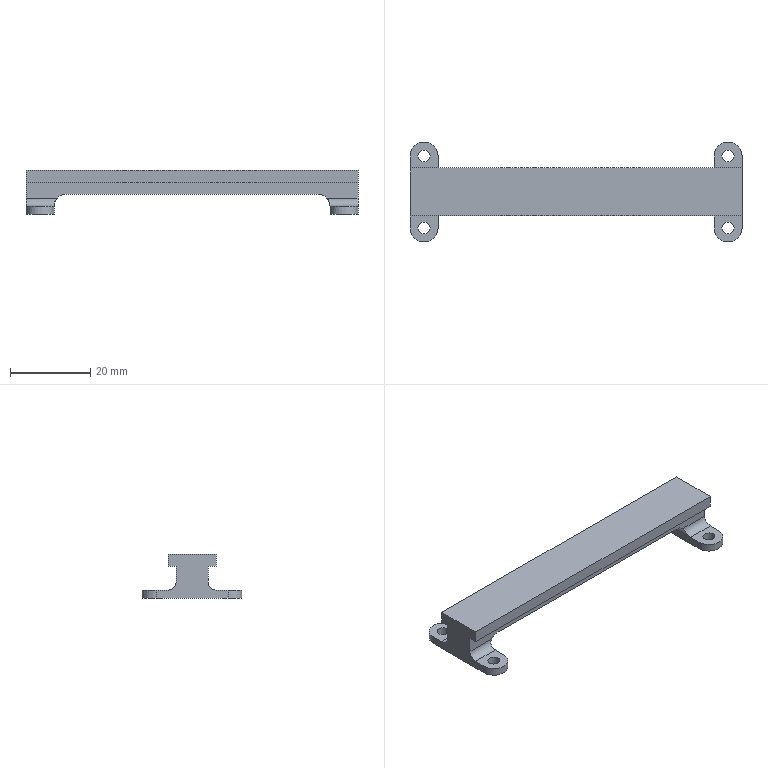Component | NX | SUPPORT_STAND | 1 solid | 32 faces | volume 5973 mm3 | plane 18 | cylinder 14 | commonest cylinder face diameters 7 x4 4 x4 3 x4 6 x2